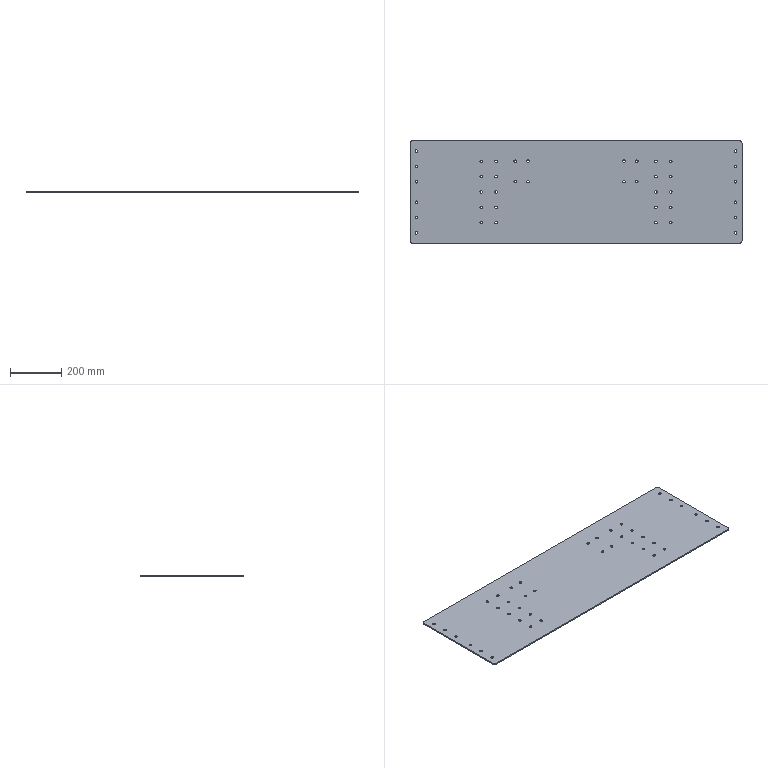Component | SolidWorks | MotorFixingPlate-1 | 1 solid | 90 faces | box 1300 x 400 x 5 mm | volume 2583863 mm3 | cylinder 84 | plane 6 | commonest cylinder face diameters 10 x80 20 x4
build123d program:
from build123d import *

# Parameters (mm, degrees)
SKETCH1_W               = 1300
SKETCH1_H               = 400
BOSS_EXTRUDE1_DEPTH     = 5
FILLET1_R               = 10
SKETCH2_R               = 5
CUT_EXTRUDE1_DEPTH      = 5
SKETCH3_R               = 5
CUT_EXTRUDE2_DEPTH      = 40
SKETCH5_R               = 5
CUT_EXTRUDE3_DEPTH      = 40
LPATTERN1_COUNT         = 5
LPATTERN1_PITCH         = 60
SKETCH7_R               = 5
CUT_EXTRUDE6_DEPTH      = 480
MIRROR3_COPY_1_SKETCH_R = 5
MIRROR3_COPY_1_DEPTH    = 5
MIRROR3_COPY_2_SKETCH_R = 5
MIRROR3_COPY_2_DEPTH    = 40
MIRROR3_COPY_3_SKETCH_R = 5
MIRROR3_COPY_3_DEPTH    = 40
MIRROR3_COPY_4_SKETCH_R = 5
MIRROR3_COPY_4_DEPTH    = 40
MIRROR3_COPY_5_SKETCH_R = 5
MIRROR3_COPY_5_DEPTH    = 40


with BuildPart() as part:
    # Sketch1 → Boss-Extrude1 (new body)
    with BuildSketch(Plane.XY):
        Rectangle(SKETCH1_W, SKETCH1_H)
    extrude(amount=BOSS_EXTRUDE1_DEPTH)

    # Fillet1
    fillet1_edges = [part.edges().sort_by_distance(p)[0] for p in [
        (650, -200, 2.5),
        (-650, -200, 2.5),
        (-650, 200, 2.5),
        (650, 200, 2.5),
    ]]
    fillet(fillet1_edges, radius=FILLET1_R)

    # Sketch2 → Cut-Extrude1 (cut)
    with BuildSketch(Plane.XY.offset(5)):
        with Locations((-625, -160)):
            Circle(SKETCH2_R)
        with Locations((-625, -100)):
            Circle(SKETCH2_R)
        with Locations((-625, -40)):
            Circle(SKETCH2_R)
    cut_extrude1 = extrude(amount=-CUT_EXTRUDE1_DEPTH, mode=Mode.SUBTRACT)

    # Mirror1: Cut-Extrude1 across plane
    add(cut_extrude1.mirror(Plane.ZX), mode=Mode.SUBTRACT)

    # Sketch3 → Cut-Extrude2 (cut)
    with BuildSketch(Plane.XY.offset(5)):
        with Locations((-371, 0)):
            Circle(SKETCH3_R)
        with Locations((-371, 60)):
            Circle(SKETCH3_R)
        with Locations((-371, 120)):
            Circle(SKETCH3_R)
        with Locations((-371, -60)):
            Circle(SKETCH3_R)
        with Locations((-371, -120)):
            Circle(SKETCH3_R)
    cut_extrude2 = extrude(amount=-CUT_EXTRUDE2_DEPTH, mode=Mode.SUBTRACT)

    # Sketch5 → Cut-Extrude3 (cut)
    with BuildSketch(Plane.XY.offset(5)):
        with Locations((-313, 120)):
            Circle(SKETCH5_R)
    cut_extrude3 = extrude(amount=-CUT_EXTRUDE3_DEPTH, mode=Mode.SUBTRACT)

    # LPattern1: Cut-Extrude3 ×5
    with Locations(*[(0, -i * LPATTERN1_PITCH, 0) for i in range(1, LPATTERN1_COUNT)]):
        add(cut_extrude3, mode=Mode.SUBTRACT)

    # Sketch7 → Cut-Extrude6 (cut)
    with BuildSketch(Plane(origin=(0, 0, 0), x_dir=(-1, 0, 0), z_dir=(0, 0, -1))):
        with Locations((238, 120.493)):
            Circle(SKETCH7_R)
        with Locations((238, 40.493)):
            Circle(SKETCH7_R)
        with Locations((188, 120.493)):
            Circle(SKETCH7_R)
        with Locations((188, 40.493)):
            Circle(SKETCH7_R)
    cut_extrude6 = extrude(amount=-CUT_EXTRUDE6_DEPTH, mode=Mode.SUBTRACT)

    # Mirror3: Cut-Extrude1, Cut-Extrude2, Cut-Extrude3, Cut-Extrude6 across plane
    add(cut_extrude1.mirror(Plane(origin=(0, 0, 0), x_dir=(0, 0, 1), z_dir=(1, 0, 0))), mode=Mode.SUBTRACT)
    add(cut_extrude2.mirror(Plane(origin=(0, 0, 0), x_dir=(0, 0, 1), z_dir=(1, 0, 0))), mode=Mode.SUBTRACT)
    add(cut_extrude3.mirror(Plane(origin=(0, 0, 0), x_dir=(0, 0, 1), z_dir=(1, 0, 0))), mode=Mode.SUBTRACT)
    add(cut_extrude6.mirror(Plane(origin=(0, 0, 0), x_dir=(0, 0, 1), z_dir=(1, 0, 0))), mode=Mode.SUBTRACT)

    # Mirror3 copy 1 sketch → Mirror3 copy 1 (cut)
    with BuildSketch(Plane(origin=(0, 0, 5), x_dir=(-1, 0, 0), z_dir=(0, 0, 1))):
        with Locations((-625, -160)):
            Circle(MIRROR3_COPY_1_SKETCH_R)
        with Locations((-625, -100)):
            Circle(MIRROR3_COPY_1_SKETCH_R)
        with Locations((-625, -40)):
            Circle(MIRROR3_COPY_1_SKETCH_R)
    extrude(amount=-MIRROR3_COPY_1_DEPTH, mode=Mode.SUBTRACT)

    # Mirror3 copy 2 sketch → Mirror3 copy 2 (cut)
    with BuildSketch(Plane(origin=(0, -60, 5), x_dir=(-1, 0, 0), z_dir=(0, 0, 1))):
        with Locations((-313, -120)):
            Circle(MIRROR3_COPY_2_SKETCH_R)
    extrude(amount=-MIRROR3_COPY_2_DEPTH, mode=Mode.SUBTRACT)

    # Mirror3 copy 3 sketch → Mirror3 copy 3 (cut)
    with BuildSketch(Plane(origin=(0, -120, 5), x_dir=(-1, 0, 0), z_dir=(0, 0, 1))):
        with Locations((-313, -120)):
            Circle(MIRROR3_COPY_3_SKETCH_R)
    extrude(amount=-MIRROR3_COPY_3_DEPTH, mode=Mode.SUBTRACT)

    # Mirror3 copy 4 sketch → Mirror3 copy 4 (cut)
    with BuildSketch(Plane(origin=(0, -180, 5), x_dir=(-1, 0, 0), z_dir=(0, 0, 1))):
        with Locations((-313, -120)):
            Circle(MIRROR3_COPY_4_SKETCH_R)
    extrude(amount=-MIRROR3_COPY_4_DEPTH, mode=Mode.SUBTRACT)

    # Mirror3 copy 5 sketch → Mirror3 copy 5 (cut)
    with BuildSketch(Plane(origin=(0, -240, 5), x_dir=(-1, 0, 0), z_dir=(0, 0, 1))):
        with Locations((-313, -120)):
            Circle(MIRROR3_COPY_5_SKETCH_R)
    extrude(amount=-MIRROR3_COPY_5_DEPTH, mode=Mode.SUBTRACT)


solid = part.part

# Placed as in the assembly
solid = solid.moved(Location((25.629, -447.9, 415), (0, 0, 0)))